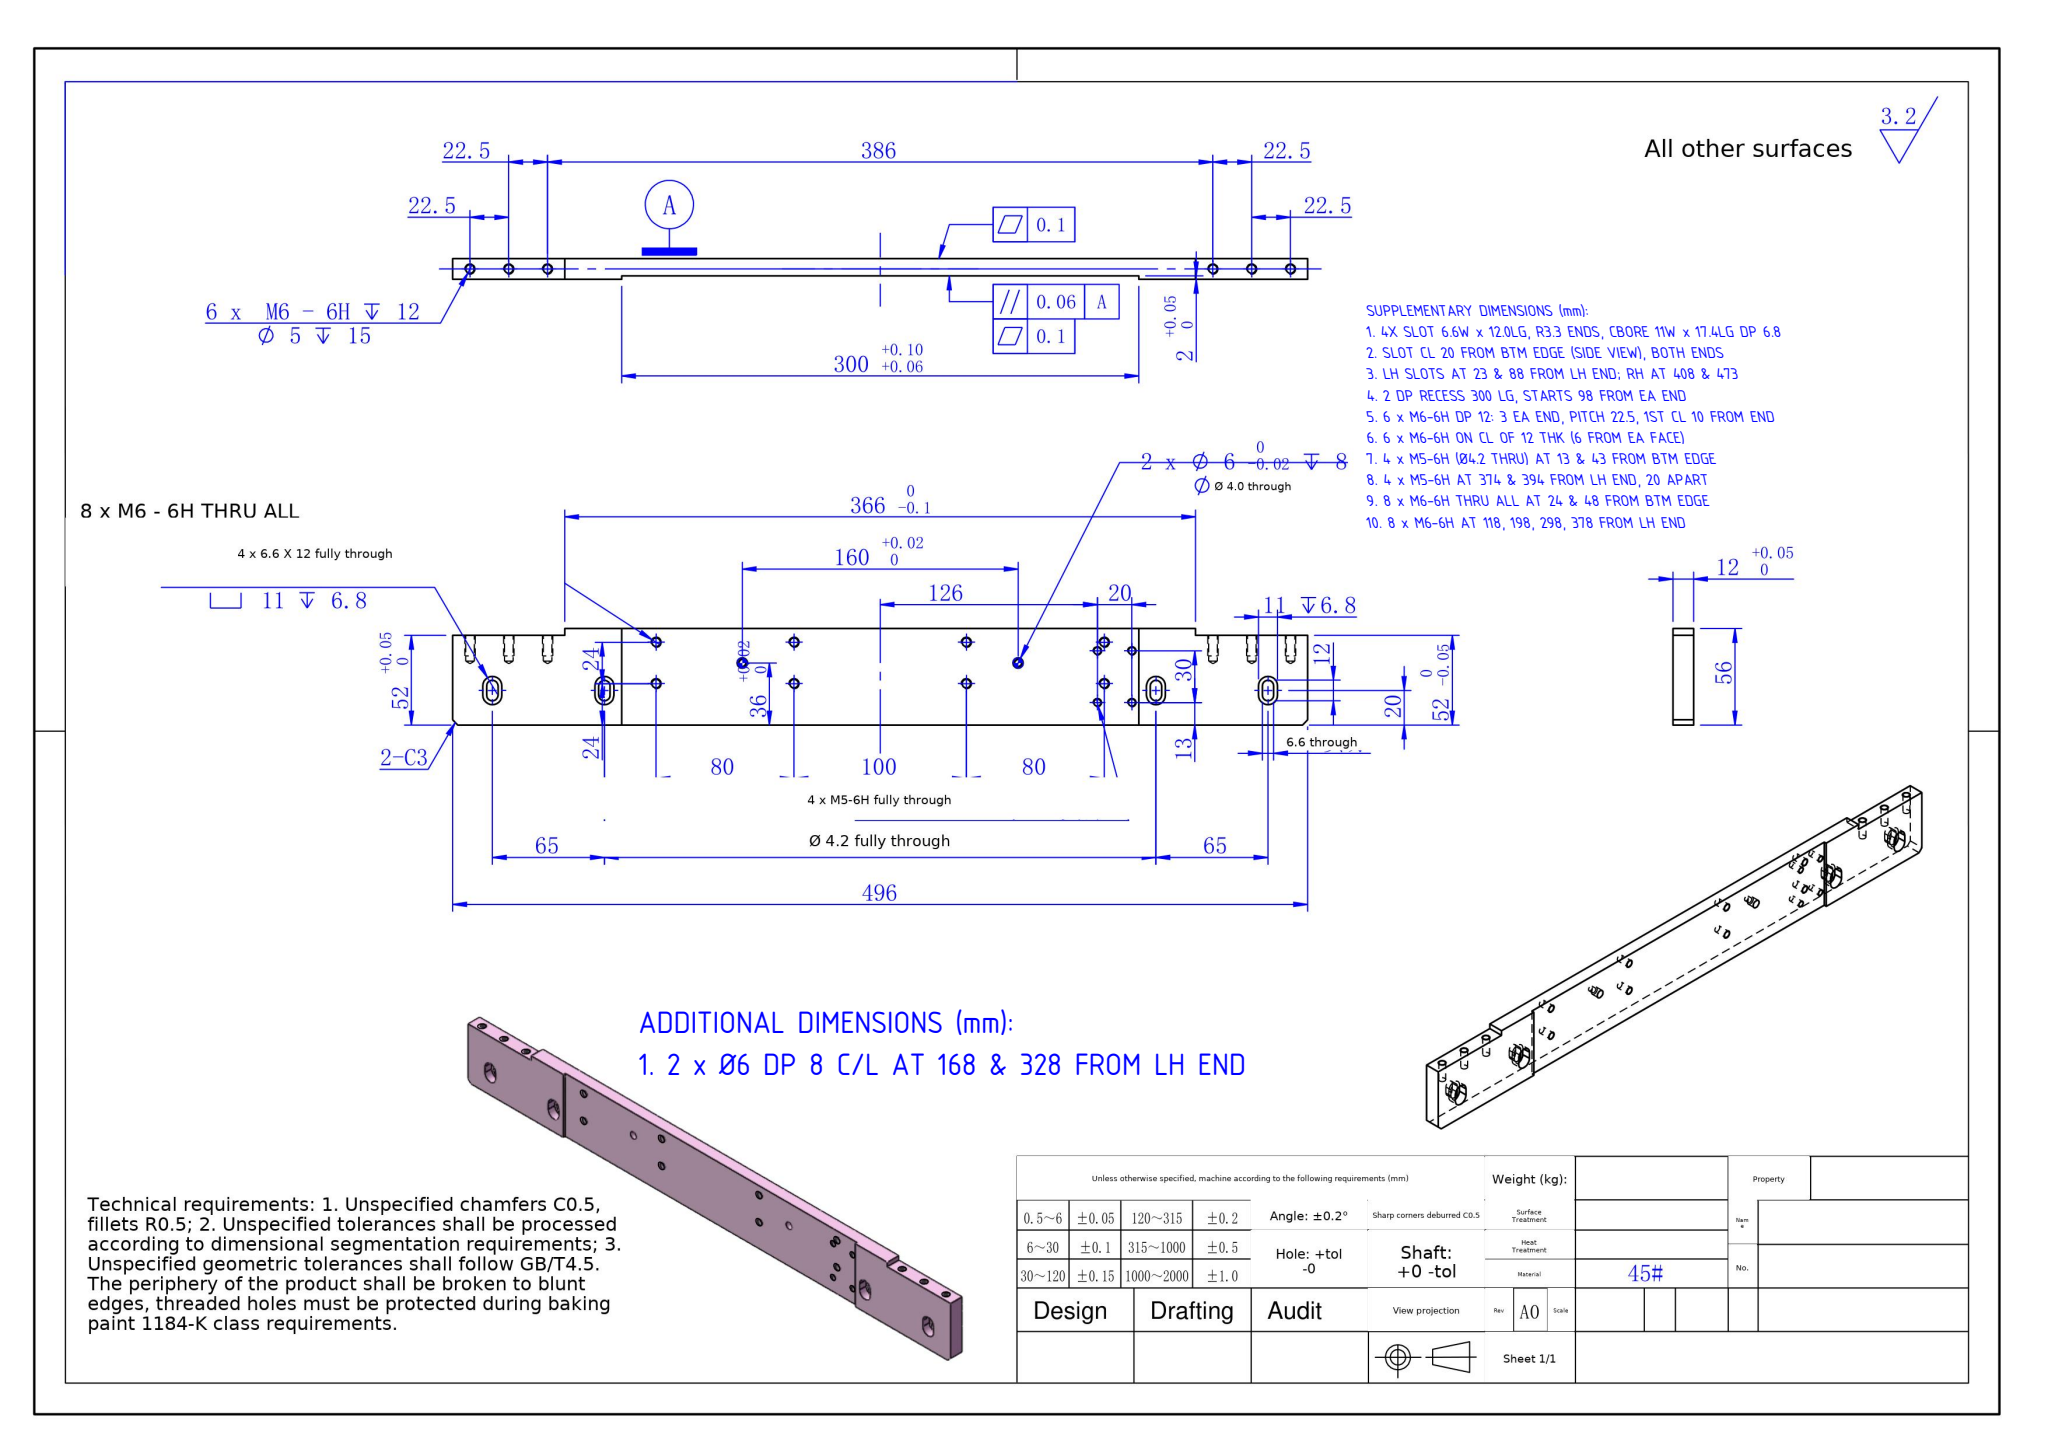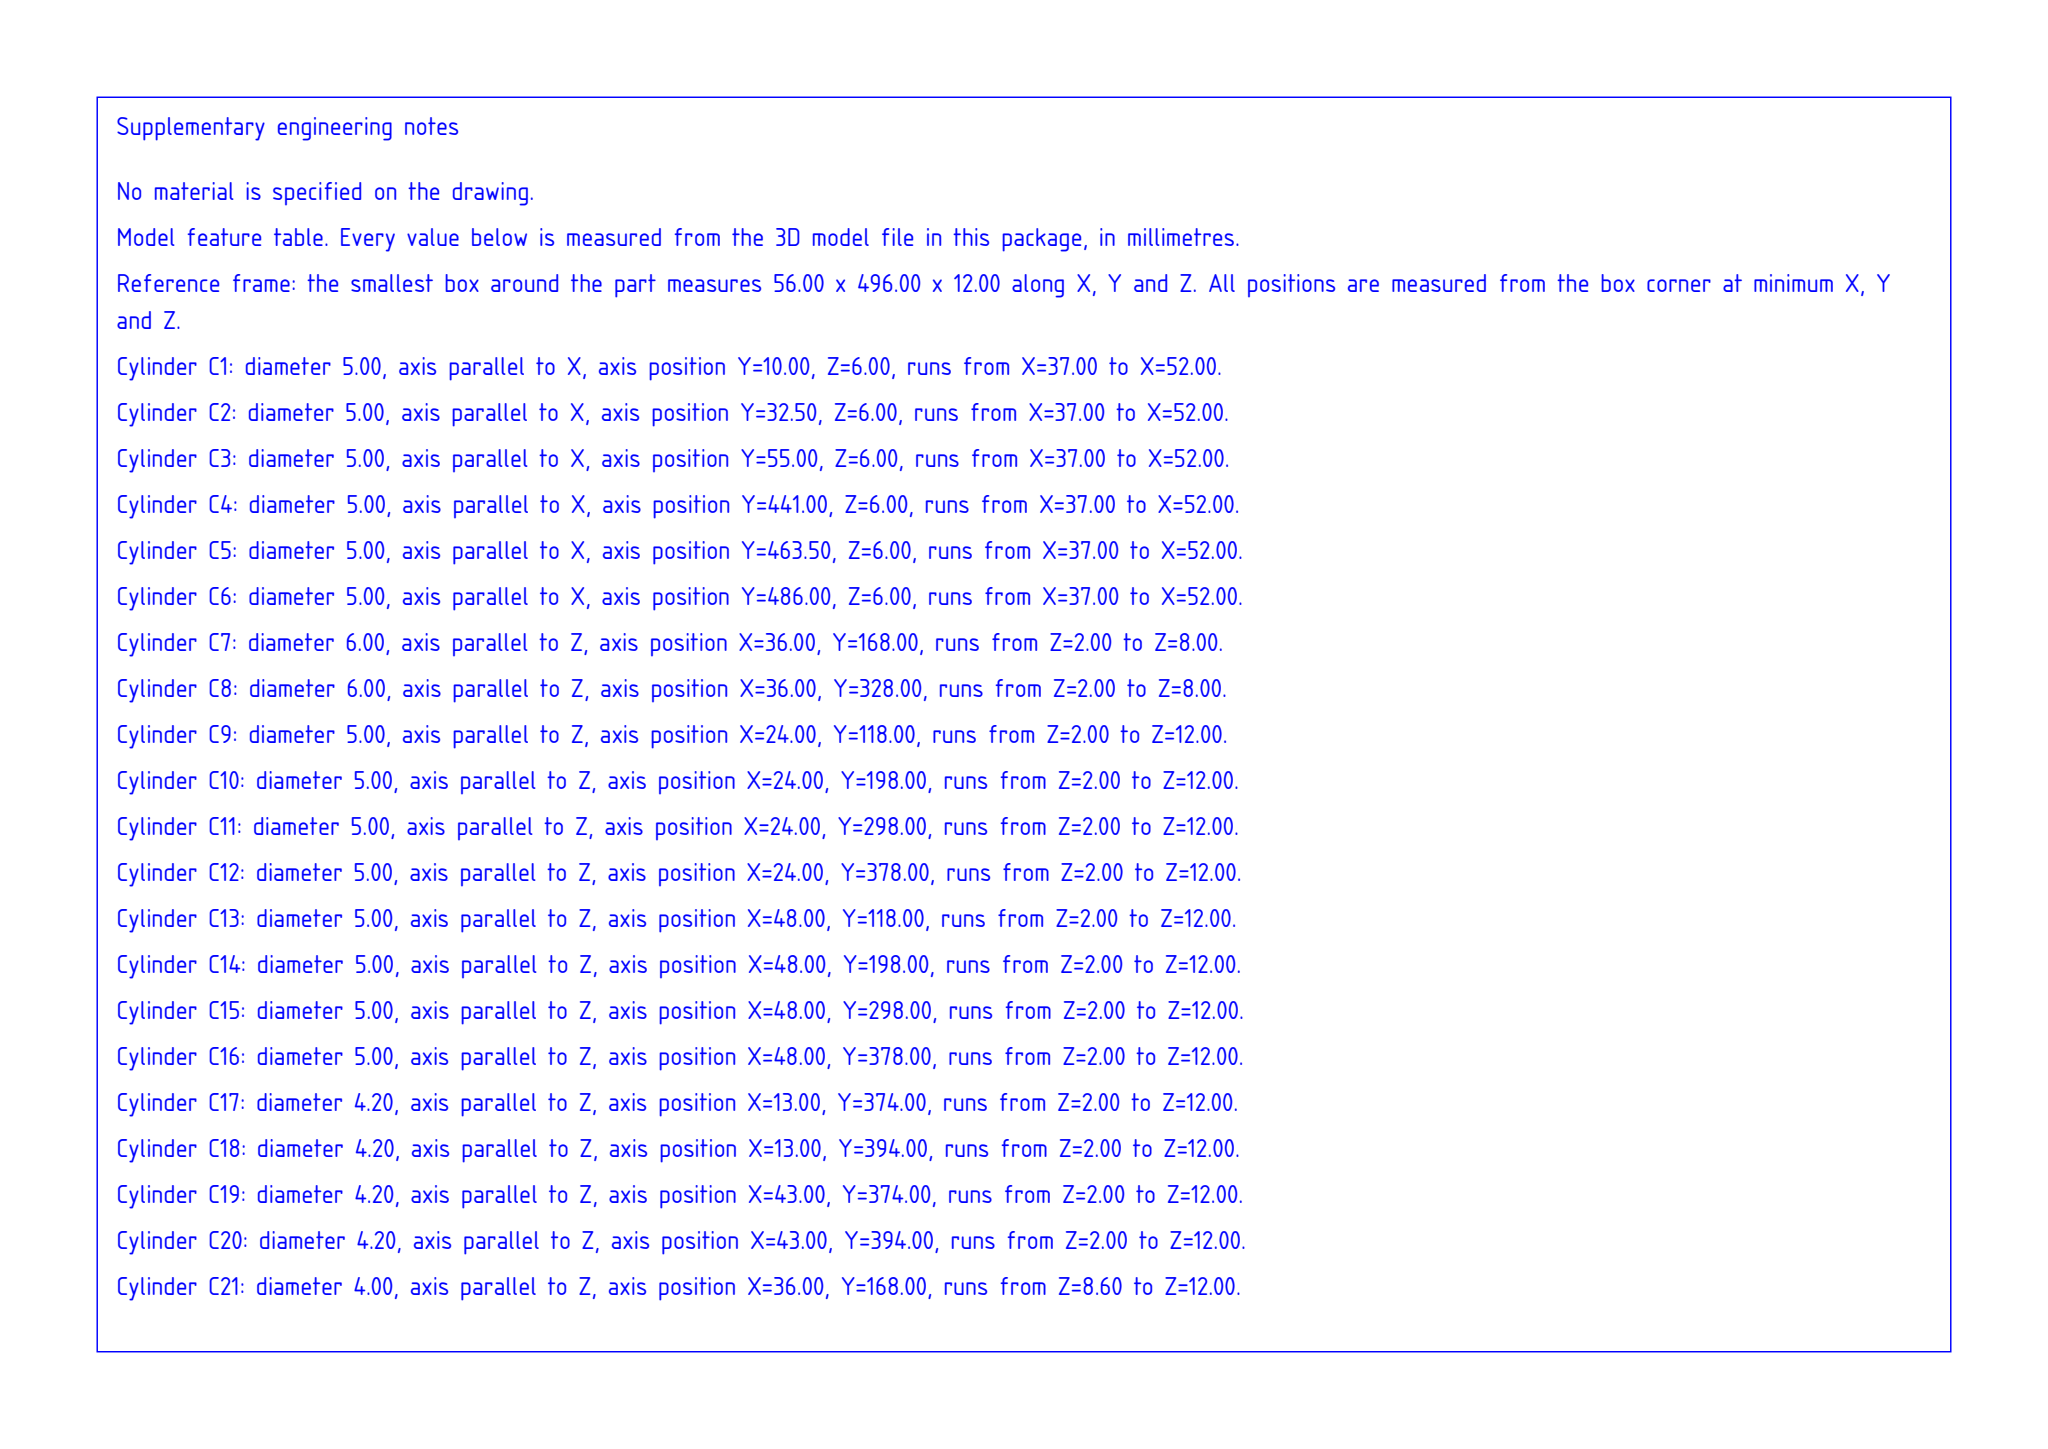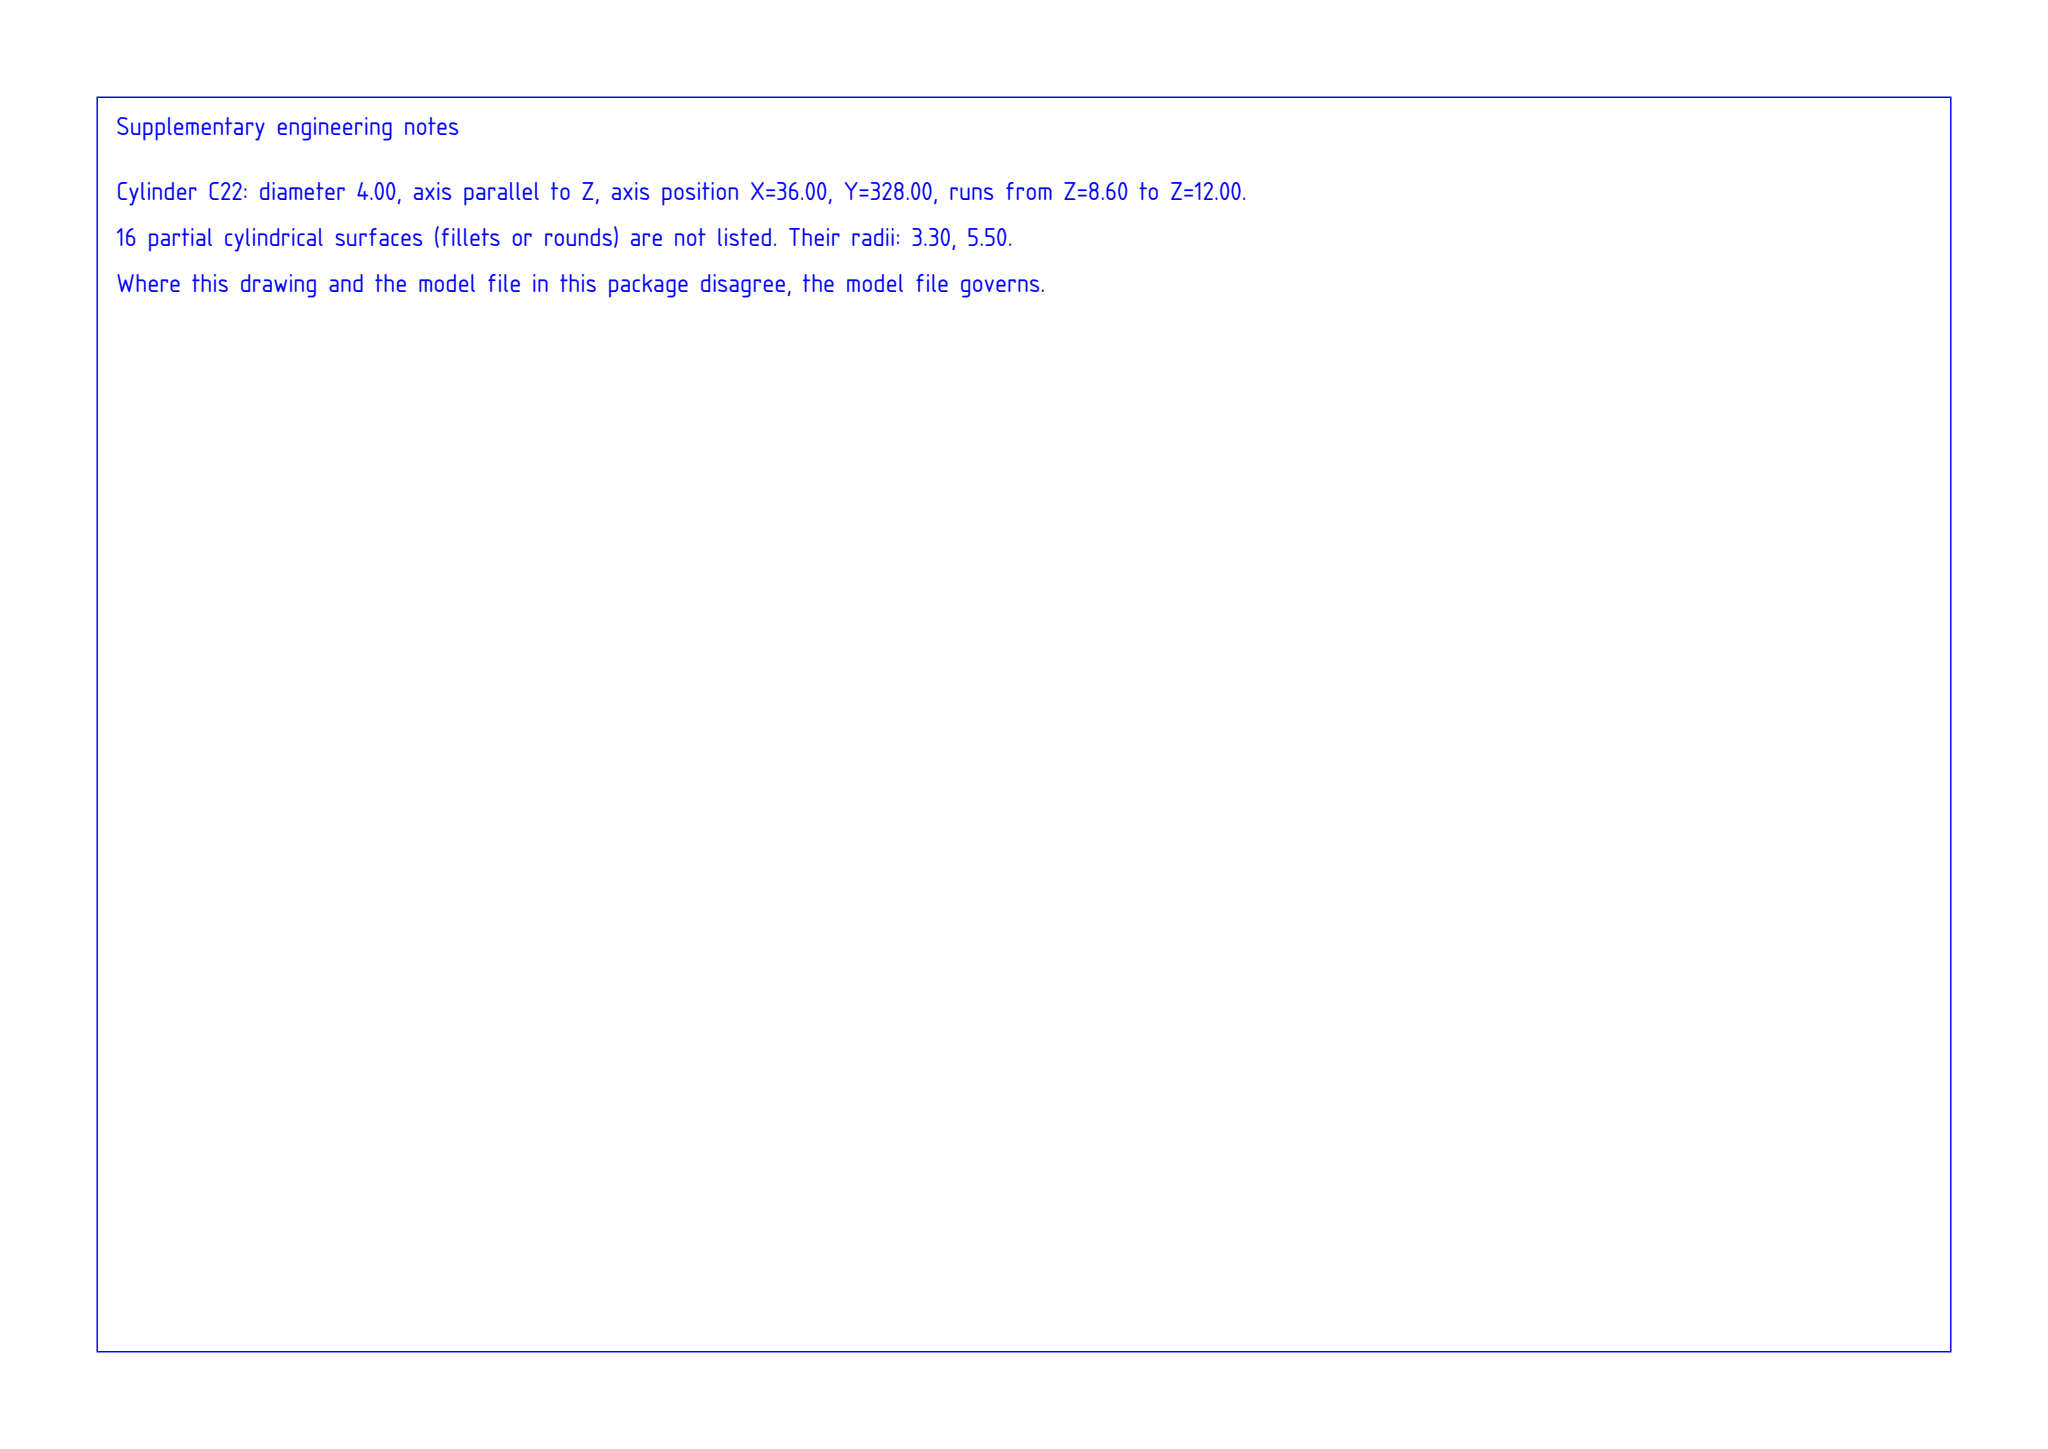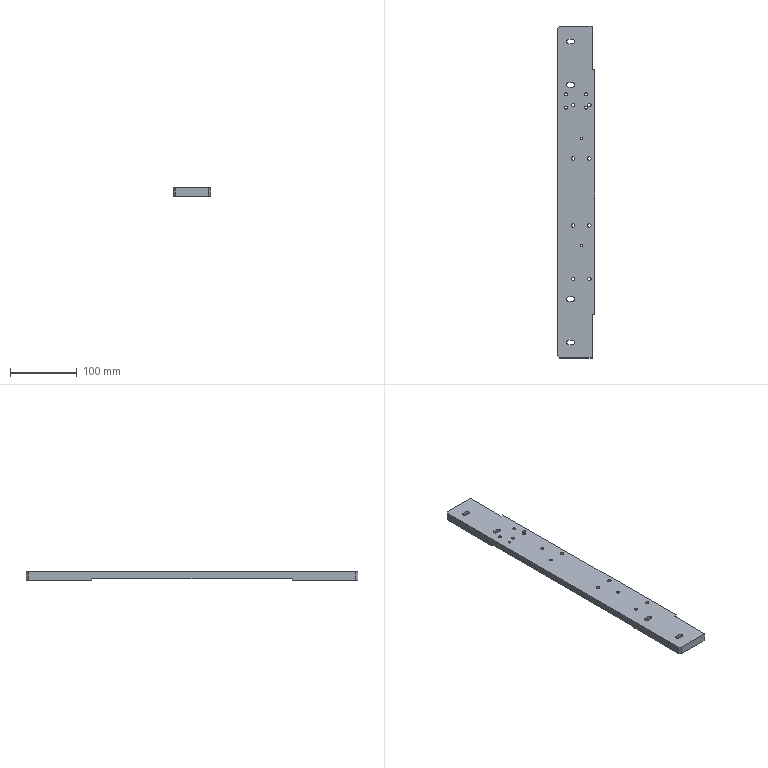Part | SolidWorks | mm | 1 solid | 120 faces | box 56 x 496 x 12 mm | volume 283311 mm3 | cylinder 68 | plane 36 | cone 16 | commonest cylinder face diameters 5 x28 11 x12 6.6 x12 4.2 x8 4 x4 6 x4